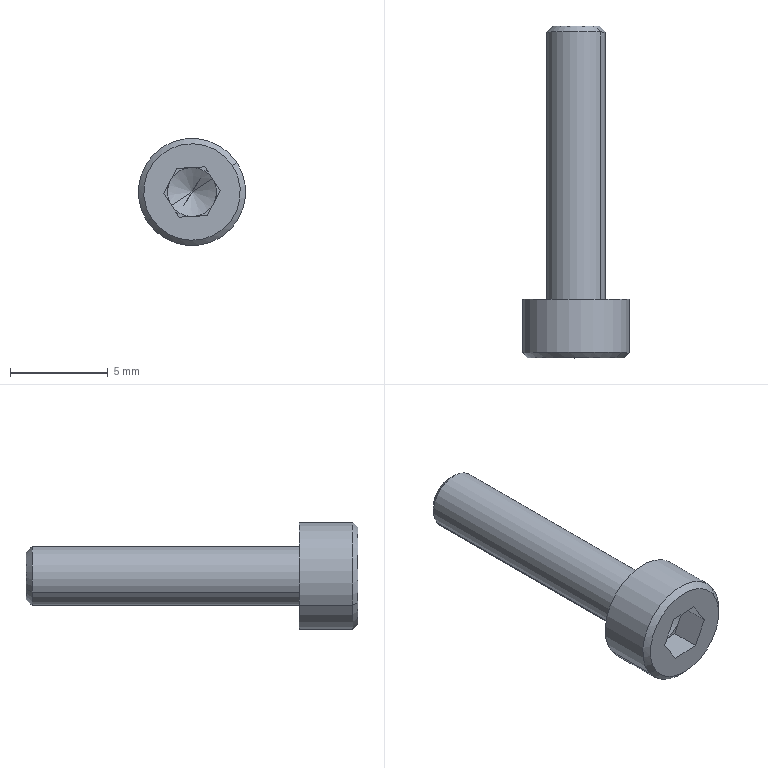Component | SolidWorks | TAC01-M3-L14-1 | 1 solid | 25 faces | box 5.5 x 17 x 5.5 mm | volume 160 mm3 | plane 15 | cone 6 | cylinder 4 | commonest cylinder face diameters 5.5 x2 3 x2
STEP:
#1=CARTESIAN_POINT('',(-2.659,1.633,8.574));
#2=VERTEX_POINT('',#1);
#3=CARTESIAN_POINT('',(-2.7,1.604,8.547));
#4=VERTEX_POINT('',#3);
#5=CARTESIAN_POINT('',(-2.659,1.633,8.574));
#6=DIRECTION('',(-0.725,-0.5,-0.4737));
#7=VECTOR('',#6,39.37);
#8=LINE('',#5,#7);
#9=EDGE_CURVE('',#2,#4,#8,.T.);
#10=ORIENTED_EDGE('',*,*,#9,.F.);
#11=CARTESIAN_POINT('',(-2.618,1.604,8.601));
#12=VERTEX_POINT('',#11);
#13=CARTESIAN_POINT('',(-2.659,1.633,8.574));
#14=DIRECTION('',(0.725,-0.5,0.4737));
#15=VECTOR('',#14,39.37);
#16=LINE('',#13,#15);
#17=EDGE_CURVE('',#2,#12,#16,.T.);
#18=ORIENTED_EDGE('',*,*,#17,.T.);
#19=CARTESIAN_POINT('',(-2.662,1.604,8.623));
#20=VERTEX_POINT('',#19);
#21=CARTESIAN_POINT('',(-2.659,1.604,8.574));
#22=DIRECTION('',(-0.,-1.,0.));
#23=DIRECTION('',(-0.8372,0.,-0.5469));
#24=AXIS2_PLACEMENT_3D('',#21,#22,#23);
#25=CIRCLE('',#24,0.04921);
#26=EDGE_CURVE('',#12,#20,#25,.T.);
#27=ORIENTED_EDGE('',*,*,#26,.T.);
#28=CARTESIAN_POINT('',(-2.703,1.604,8.597));
#29=VERTEX_POINT('',#28);
#30=CARTESIAN_POINT('',(-2.659,1.604,8.574));
#31=DIRECTION('',(-0.,-1.,0.));
#32=DIRECTION('',(-0.8372,0.,-0.5469));
#33=AXIS2_PLACEMENT_3D('',#30,#31,#32);
#34=CIRCLE('',#33,0.04921);
#35=EDGE_CURVE('',#20,#29,#34,.T.);
#36=ORIENTED_EDGE('',*,*,#35,.T.);
#37=CARTESIAN_POINT('',(-2.659,1.604,8.574));
#38=DIRECTION('',(-0.,-1.,0.));
#39=DIRECTION('',(-0.8372,0.,-0.5469));
#40=AXIS2_PLACEMENT_3D('',#37,#38,#39);
#41=CIRCLE('',#40,0.04921);
#42=EDGE_CURVE('',#29,#4,#41,.T.);
#43=ORIENTED_EDGE('',*,*,#42,.T.);
#44=EDGE_LOOP('',(#10,#18,#27,#36,#43));
#45=FACE_OUTER_BOUND('',#44,.T.);
#46=CARTESIAN_POINT('',(-2.659,-37.737,8.574));
#47=DIRECTION('',(-0.,-1.,0.));
#48=DIRECTION('',(-0.8372,0.,-0.5469));
#49=AXIS2_PLACEMENT_3D('',#46,#47,#48);
#50=CONICAL_SURFACE('',#49,68.191,1.047);
#51=ADVANCED_FACE('',(#45),#50,.F.);
#52=CARTESIAN_POINT('',(-2.75,1.663,8.515));
#53=VERTEX_POINT('',#52);
#54=CARTESIAN_POINT('',(-2.568,1.663,8.634));
#55=VERTEX_POINT('',#54);
#56=CARTESIAN_POINT('',(-2.659,1.663,8.574));
#57=DIRECTION('',(-0.,-1.,0.));
#58=DIRECTION('',(-0.8372,0.,-0.5469));
#59=AXIS2_PLACEMENT_3D('',#56,#57,#58);
#60=CIRCLE('',#59,0.1083);
#61=EDGE_CURVE('',#53,#55,#60,.T.);
#62=ORIENTED_EDGE('',*,*,#61,.T.);
#63=CARTESIAN_POINT('',(-2.568,1.556,8.634));
#64=VERTEX_POINT('',#63);
#65=CARTESIAN_POINT('',(-2.568,1.663,8.634));
#66=DIRECTION('',(-0.,-1.,0.));
#67=VECTOR('',#66,39.37);
#68=LINE('',#65,#67);
#69=EDGE_CURVE('',#55,#64,#68,.T.);
#70=ORIENTED_EDGE('',*,*,#69,.T.);
#71=CARTESIAN_POINT('',(-2.75,1.556,8.515));
#72=VERTEX_POINT('',#71);
#73=CARTESIAN_POINT('',(-2.659,1.556,8.574));
#74=DIRECTION('',(-0.,-1.,0.));
#75=DIRECTION('',(-0.8372,0.,-0.5469));
#76=AXIS2_PLACEMENT_3D('',#73,#74,#75);
#77=CIRCLE('',#76,0.1083);
#78=EDGE_CURVE('',#72,#64,#77,.T.);
#79=ORIENTED_EDGE('',*,*,#78,.F.);
#80=CARTESIAN_POINT('',(-2.75,1.663,8.515));
#81=DIRECTION('',(-0.,-1.,0.));
#82=VECTOR('',#81,39.37);
#83=LINE('',#80,#82);
#84=EDGE_CURVE('',#53,#72,#83,.T.);
#85=ORIENTED_EDGE('',*,*,#84,.F.);
#86=EDGE_LOOP('',(#62,#70,#79,#85));
#87=FACE_OUTER_BOUND('',#86,.T.);
#88=CARTESIAN_POINT('',(-2.659,1.663,8.574));
#89=DIRECTION('',(-0.,-1.,0.));
#90=DIRECTION('',(-0.8372,0.,-0.5469));
#91=AXIS2_PLACEMENT_3D('',#88,#89,#90);
#92=CYLINDRICAL_SURFACE('',#91,0.1083);
#93=ADVANCED_FACE('',(#87),#92,.T.);
#94=CARTESIAN_POINT('',(-2.74,1.545,8.521));
#95=VERTEX_POINT('',#94);
#96=CARTESIAN_POINT('',(-2.577,1.545,8.628));
#97=VERTEX_POINT('',#96);
#98=CARTESIAN_POINT('',(-2.659,1.545,8.574));
#99=DIRECTION('',(-0.,-1.,0.));
#100=DIRECTION('',(-0.8372,0.,-0.5469));
#101=AXIS2_PLACEMENT_3D('',#98,#99,#100);
#102=CIRCLE('',#101,0.09744);
#103=EDGE_CURVE('',#95,#97,#102,.T.);
#104=ORIENTED_EDGE('',*,*,#103,.F.);
#105=CARTESIAN_POINT('',(-2.75,1.556,8.515));
#106=DIRECTION('',(-0.592,0.7071,-0.3867));
#107=VECTOR('',#106,39.37);
#108=LINE('',#105,#107);
#109=EDGE_CURVE('',#95,#72,#108,.T.);
#110=ORIENTED_EDGE('',*,*,#109,.T.);
#111=ORIENTED_EDGE('',*,*,#78,.T.);
#112=CARTESIAN_POINT('',(-2.568,1.556,8.634));
#113=DIRECTION('',(0.592,0.7071,0.3867));
#114=VECTOR('',#113,39.37);
#115=LINE('',#112,#114);
#116=EDGE_CURVE('',#97,#64,#115,.T.);
#117=ORIENTED_EDGE('',*,*,#116,.F.);
#118=EDGE_LOOP('',(#104,#110,#111,#117));
#119=FACE_OUTER_BOUND('',#118,.T.);
#120=CARTESIAN_POINT('',(-2.659,1.556,8.574));
#121=DIRECTION('',(0.,1.,-0.));
#122=DIRECTION('',(0.8372,-0.,0.5469));
#123=AXIS2_PLACEMENT_3D('',#120,#121,#122);
#124=CONICAL_SURFACE('',#123,0.1083,0.7854);
#125=ADVANCED_FACE('',(#119),#124,.T.);
#126=CARTESIAN_POINT('',(-2.698,2.215,8.549));
#127=VERTEX_POINT('',#126);
#128=CARTESIAN_POINT('',(-2.62,2.215,8.6));
#129=VERTEX_POINT('',#128);
#130=CARTESIAN_POINT('',(-2.659,2.215,8.574));
#131=DIRECTION('',(-0.,-1.,0.));
#132=DIRECTION('',(-0.8372,0.,-0.5469));
#133=AXIS2_PLACEMENT_3D('',#130,#131,#132);
#134=CIRCLE('',#133,0.04699);
#135=EDGE_CURVE('',#127,#129,#134,.T.);
#136=ORIENTED_EDGE('',*,*,#135,.T.);
#137=CARTESIAN_POINT('',(-2.609,2.202,8.607));
#138=VERTEX_POINT('',#137);
#139=CARTESIAN_POINT('',(-2.62,2.215,8.6));
#140=DIRECTION('',(0.592,-0.7071,0.3867));
#141=VECTOR('',#140,39.37);
#142=LINE('',#139,#141);
#143=EDGE_CURVE('',#129,#138,#142,.T.);
#144=ORIENTED_EDGE('',*,*,#143,.T.);
#145=CARTESIAN_POINT('',(-2.708,2.202,8.542));
#146=VERTEX_POINT('',#145);
#147=CARTESIAN_POINT('',(-2.659,2.202,8.574));
#148=DIRECTION('',(-0.,-1.,0.));
#149=DIRECTION('',(-0.8372,0.,-0.5469));
#150=AXIS2_PLACEMENT_3D('',#147,#148,#149);
#151=CIRCLE('',#150,0.05906);
#152=EDGE_CURVE('',#146,#138,#151,.T.);
#153=ORIENTED_EDGE('',*,*,#152,.F.);
#154=CARTESIAN_POINT('',(-2.698,2.215,8.549));
#155=DIRECTION('',(-0.592,-0.7071,-0.3867));
#156=VECTOR('',#155,39.37);
#157=LINE('',#154,#156);
#158=EDGE_CURVE('',#127,#146,#157,.T.);
#159=ORIENTED_EDGE('',*,*,#158,.F.);
#160=EDGE_LOOP('',(#136,#144,#153,#159));
#161=FACE_OUTER_BOUND('',#160,.T.);
#162=CARTESIAN_POINT('',(-2.659,2.215,8.574));
#163=DIRECTION('',(-0.,-1.,0.));
#164=DIRECTION('',(-0.8372,0.,-0.5469));
#165=AXIS2_PLACEMENT_3D('',#162,#163,#164);
#166=CONICAL_SURFACE('',#165,0.04699,0.7854);
#167=ADVANCED_FACE('',(#161),#166,.T.);
#168=ORIENTED_EDGE('',*,*,#152,.T.);
#169=CARTESIAN_POINT('',(-2.609,1.663,8.607));
#170=VERTEX_POINT('',#169);
#171=CARTESIAN_POINT('',(-2.609,2.215,8.607));
#172=DIRECTION('',(-0.,-1.,0.));
#173=VECTOR('',#172,39.37);
#174=LINE('',#171,#173);
#175=EDGE_CURVE('',#138,#170,#174,.T.);
#176=ORIENTED_EDGE('',*,*,#175,.T.);
#177=CARTESIAN_POINT('',(-2.708,1.663,8.542));
#178=VERTEX_POINT('',#177);
#179=CARTESIAN_POINT('',(-2.659,1.663,8.574));
#180=DIRECTION('',(-0.,-1.,0.));
#181=DIRECTION('',(-0.8372,0.,-0.5469));
#182=AXIS2_PLACEMENT_3D('',#179,#180,#181);
#183=CIRCLE('',#182,0.05906);
#184=EDGE_CURVE('',#178,#170,#183,.T.);
#185=ORIENTED_EDGE('',*,*,#184,.F.);
#186=CARTESIAN_POINT('',(-2.708,2.215,8.542));
#187=DIRECTION('',(-0.,-1.,0.));
#188=VECTOR('',#187,39.37);
#189=LINE('',#186,#188);
#190=EDGE_CURVE('',#146,#178,#189,.T.);
#191=ORIENTED_EDGE('',*,*,#190,.F.);
#192=EDGE_LOOP('',(#168,#176,#185,#191));
#193=FACE_OUTER_BOUND('',#192,.T.);
#194=CARTESIAN_POINT('',(-2.659,2.215,8.574));
#195=DIRECTION('',(-0.,-1.,0.));
#196=DIRECTION('',(-0.8372,0.,-0.5469));
#197=AXIS2_PLACEMENT_3D('',#194,#195,#196);
#198=CYLINDRICAL_SURFACE('',#197,0.05906);
#199=ADVANCED_FACE('',(#193),#198,.T.);
#200=CARTESIAN_POINT('',(-2.656,1.604,8.525));
#201=VERTEX_POINT('',#200);
#202=CARTESIAN_POINT('',(-2.659,1.604,8.574));
#203=DIRECTION('',(-0.,-1.,0.));
#204=DIRECTION('',(-0.8372,0.,-0.5469));
#205=AXIS2_PLACEMENT_3D('',#202,#203,#204);
#206=CIRCLE('',#205,0.04921);
#207=EDGE_CURVE('',#4,#201,#206,.T.);
#208=ORIENTED_EDGE('',*,*,#207,.F.);
#209=CARTESIAN_POINT('',(-2.685,1.604,8.524));
#210=VERTEX_POINT('',#209);
#211=CARTESIAN_POINT('',(-2.716,1.604,8.571));
#212=DIRECTION('',(0.5469,-0.,-0.8372));
#213=VECTOR('',#212,39.37);
#214=LINE('',#211,#213);
#215=EDGE_CURVE('',#4,#210,#214,.T.);
#216=ORIENTED_EDGE('',*,*,#215,.T.);
#217=CARTESIAN_POINT('',(-2.685,1.604,8.524));
#218=DIRECTION('',(0.9985,-0.,0.05508));
#219=VECTOR('',#218,39.37);
#220=LINE('',#217,#219);
#221=EDGE_CURVE('',#210,#201,#220,.T.);
#222=ORIENTED_EDGE('',*,*,#221,.T.);
#223=EDGE_LOOP('',(#208,#216,#222));
#224=FACE_OUTER_BOUND('',#223,.T.);
#225=CARTESIAN_POINT('',(-2.659,1.604,8.574));
#226=DIRECTION('',(-0.,-1.,0.));
#227=DIRECTION('',(-0.8372,0.,-0.5469));
#228=AXIS2_PLACEMENT_3D('',#225,#226,#227);
#229=PLANE('',#228);
#230=ADVANCED_FACE('',(#224),#229,.T.);
#231=CARTESIAN_POINT('',(-2.615,1.604,8.552));
#232=VERTEX_POINT('',#231);
#233=CARTESIAN_POINT('',(-2.659,1.604,8.574));
#234=DIRECTION('',(-0.,-1.,0.));
#235=DIRECTION('',(-0.8372,0.,-0.5469));
#236=AXIS2_PLACEMENT_3D('',#233,#234,#235);
#237=CIRCLE('',#236,0.04921);
#238=EDGE_CURVE('',#201,#232,#237,.T.);
#239=ORIENTED_EDGE('',*,*,#238,.F.);
#240=CARTESIAN_POINT('',(-2.628,1.604,8.527));
#241=VERTEX_POINT('',#240);
#242=CARTESIAN_POINT('',(-2.685,1.604,8.524));
#243=DIRECTION('',(0.9985,-0.,0.05508));
#244=VECTOR('',#243,39.37);
#245=LINE('',#242,#244);
#246=EDGE_CURVE('',#201,#241,#245,.T.);
#247=ORIENTED_EDGE('',*,*,#246,.T.);
#248=CARTESIAN_POINT('',(-2.628,1.604,8.527));
#249=DIRECTION('',(0.4515,-0.,0.8923));
#250=VECTOR('',#249,39.37);
#251=LINE('',#248,#250);
#252=EDGE_CURVE('',#241,#232,#251,.T.);
#253=ORIENTED_EDGE('',*,*,#252,.T.);
#254=EDGE_LOOP('',(#239,#247,#253));
#255=FACE_OUTER_BOUND('',#254,.T.);
#256=CARTESIAN_POINT('',(-2.659,1.604,8.574));
#257=DIRECTION('',(-0.,-1.,0.));
#258=DIRECTION('',(-0.8372,0.,-0.5469));
#259=AXIS2_PLACEMENT_3D('',#256,#257,#258);
#260=PLANE('',#259);
#261=ADVANCED_FACE('',(#255),#260,.T.);
#262=CARTESIAN_POINT('',(-2.659,1.604,8.574));
#263=DIRECTION('',(-0.,-1.,0.));
#264=DIRECTION('',(-0.8372,0.,-0.5469));
#265=AXIS2_PLACEMENT_3D('',#262,#263,#264);
#266=CIRCLE('',#265,0.04921);
#267=EDGE_CURVE('',#232,#12,#266,.T.);
#268=ORIENTED_EDGE('',*,*,#267,.F.);
#269=CARTESIAN_POINT('',(-2.602,1.604,8.577));
#270=VERTEX_POINT('',#269);
#271=CARTESIAN_POINT('',(-2.628,1.604,8.527));
#272=DIRECTION('',(0.4515,-0.,0.8923));
#273=VECTOR('',#272,39.37);
#274=LINE('',#271,#273);
#275=EDGE_CURVE('',#232,#270,#274,.T.);
#276=ORIENTED_EDGE('',*,*,#275,.T.);
#277=CARTESIAN_POINT('',(-2.602,1.604,8.577));
#278=DIRECTION('',(-0.5469,0.,0.8372));
#279=VECTOR('',#278,39.37);
#280=LINE('',#277,#279);
#281=EDGE_CURVE('',#270,#12,#280,.T.);
#282=ORIENTED_EDGE('',*,*,#281,.T.);
#283=EDGE_LOOP('',(#268,#276,#282));
#284=FACE_OUTER_BOUND('',#283,.T.);
#285=CARTESIAN_POINT('',(-2.659,1.604,8.574));
#286=DIRECTION('',(-0.,-1.,0.));
#287=DIRECTION('',(-0.8372,0.,-0.5469));
#288=AXIS2_PLACEMENT_3D('',#285,#286,#287);
#289=PLANE('',#288);
#290=ADVANCED_FACE('',(#284),#289,.T.);
#291=ORIENTED_EDGE('',*,*,#26,.F.);
#292=CARTESIAN_POINT('',(-2.633,1.604,8.625));
#293=VERTEX_POINT('',#292);
#294=CARTESIAN_POINT('',(-2.602,1.604,8.577));
#295=DIRECTION('',(-0.5469,0.,0.8372));
#296=VECTOR('',#295,39.37);
#297=LINE('',#294,#296);
#298=EDGE_CURVE('',#12,#293,#297,.T.);
#299=ORIENTED_EDGE('',*,*,#298,.T.);
#300=CARTESIAN_POINT('',(-2.633,1.604,8.625));
#301=DIRECTION('',(-0.9985,0.,-0.05508));
#302=VECTOR('',#301,39.37);
#303=LINE('',#300,#302);
#304=EDGE_CURVE('',#293,#20,#303,.T.);
#305=ORIENTED_EDGE('',*,*,#304,.T.);
#306=EDGE_LOOP('',(#291,#299,#305));
#307=FACE_OUTER_BOUND('',#306,.T.);
#308=CARTESIAN_POINT('',(-2.659,1.604,8.574));
#309=DIRECTION('',(-0.,-1.,0.));
#310=DIRECTION('',(-0.8372,0.,-0.5469));
#311=AXIS2_PLACEMENT_3D('',#308,#309,#310);
#312=PLANE('',#311);
#313=ADVANCED_FACE('',(#307),#312,.T.);
#314=ORIENTED_EDGE('',*,*,#35,.F.);
#315=CARTESIAN_POINT('',(-2.69,1.604,8.622));
#316=VERTEX_POINT('',#315);
#317=CARTESIAN_POINT('',(-2.633,1.604,8.625));
#318=DIRECTION('',(-0.9985,0.,-0.05508));
#319=VECTOR('',#318,39.37);
#320=LINE('',#317,#319);
#321=EDGE_CURVE('',#20,#316,#320,.T.);
#322=ORIENTED_EDGE('',*,*,#321,.T.);
#323=CARTESIAN_POINT('',(-2.69,1.604,8.622));
#324=DIRECTION('',(-0.4515,0.,-0.8923));
#325=VECTOR('',#324,39.37);
#326=LINE('',#323,#325);
#327=EDGE_CURVE('',#316,#29,#326,.T.);
#328=ORIENTED_EDGE('',*,*,#327,.T.);
#329=EDGE_LOOP('',(#314,#322,#328));
#330=FACE_OUTER_BOUND('',#329,.T.);
#331=CARTESIAN_POINT('',(-2.659,1.604,8.574));
#332=DIRECTION('',(-0.,-1.,0.));
#333=DIRECTION('',(-0.8372,0.,-0.5469));
#334=AXIS2_PLACEMENT_3D('',#331,#332,#333);
#335=PLANE('',#334);
#336=ADVANCED_FACE('',(#330),#335,.T.);
#337=ORIENTED_EDGE('',*,*,#175,.F.);
#338=CARTESIAN_POINT('',(-2.659,2.202,8.574));
#339=DIRECTION('',(-0.,-1.,0.));
#340=DIRECTION('',(-0.8372,0.,-0.5469));
#341=AXIS2_PLACEMENT_3D('',#338,#339,#340);
#342=CIRCLE('',#341,0.05906);
#343=EDGE_CURVE('',#138,#146,#342,.T.);
#344=ORIENTED_EDGE('',*,*,#343,.T.);
#345=ORIENTED_EDGE('',*,*,#190,.T.);
#346=CARTESIAN_POINT('',(-2.659,1.663,8.574));
#347=DIRECTION('',(-0.,-1.,0.));
#348=DIRECTION('',(-0.8372,0.,-0.5469));
#349=AXIS2_PLACEMENT_3D('',#346,#347,#348);
#350=CIRCLE('',#349,0.05906);
#351=EDGE_CURVE('',#170,#178,#350,.T.);
#352=ORIENTED_EDGE('',*,*,#351,.F.);
#353=EDGE_LOOP('',(#337,#344,#345,#352));
#354=FACE_OUTER_BOUND('',#353,.T.);
#355=CARTESIAN_POINT('',(-2.659,2.215,8.574));
#356=DIRECTION('',(-0.,-1.,0.));
#357=DIRECTION('',(-0.8372,0.,-0.5469));
#358=AXIS2_PLACEMENT_3D('',#355,#356,#357);
#359=CYLINDRICAL_SURFACE('',#358,0.05906);
#360=ADVANCED_FACE('',(#354),#359,.T.);
#361=ORIENTED_EDGE('',*,*,#143,.F.);
#362=CARTESIAN_POINT('',(-2.659,2.215,8.574));
#363=DIRECTION('',(-0.,-1.,0.));
#364=DIRECTION('',(-0.8372,0.,-0.5469));
#365=AXIS2_PLACEMENT_3D('',#362,#363,#364);
#366=CIRCLE('',#365,0.04699);
#367=EDGE_CURVE('',#129,#127,#366,.T.);
#368=ORIENTED_EDGE('',*,*,#367,.T.);
#369=ORIENTED_EDGE('',*,*,#158,.T.);
#370=ORIENTED_EDGE('',*,*,#343,.F.);
#371=EDGE_LOOP('',(#361,#368,#369,#370));
#372=FACE_OUTER_BOUND('',#371,.T.);
#373=CARTESIAN_POINT('',(-2.659,2.215,8.574));
#374=DIRECTION('',(-0.,-1.,0.));
#375=DIRECTION('',(-0.8372,0.,-0.5469));
#376=AXIS2_PLACEMENT_3D('',#373,#374,#375);
#377=CONICAL_SURFACE('',#376,0.04699,0.7854);
#378=ADVANCED_FACE('',(#372),#377,.T.);
#379=ORIENTED_EDGE('',*,*,#135,.F.);
#380=ORIENTED_EDGE('',*,*,#367,.F.);
#381=EDGE_LOOP('',(#379,#380));
#382=FACE_OUTER_BOUND('',#381,.T.);
#383=CARTESIAN_POINT('',(-2.633,2.215,8.535));
#384=DIRECTION('',(-0.,-1.,0.));
#385=DIRECTION('',(-0.8372,0.,-0.5469));
#386=AXIS2_PLACEMENT_3D('',#383,#384,#385);
#387=PLANE('',#386);
#388=ADVANCED_FACE('',(#382),#387,.F.);
#389=CARTESIAN_POINT('',(-2.69,1.545,8.622));
#390=VERTEX_POINT('',#389);
#391=CARTESIAN_POINT('',(-2.716,1.545,8.571));
#392=VERTEX_POINT('',#391);
#393=CARTESIAN_POINT('',(-2.69,1.545,8.622));
#394=DIRECTION('',(-0.4515,0.,-0.8923));
#395=VECTOR('',#394,39.37);
#396=LINE('',#393,#395);
#397=EDGE_CURVE('',#390,#392,#396,.T.);
#398=ORIENTED_EDGE('',*,*,#397,.F.);
#399=CARTESIAN_POINT('',(-2.633,1.545,8.625));
#400=VERTEX_POINT('',#399);
#401=CARTESIAN_POINT('',(-2.633,1.545,8.625));
#402=DIRECTION('',(-0.9985,0.,-0.05508));
#403=VECTOR('',#402,39.37);
#404=LINE('',#401,#403);
#405=EDGE_CURVE('',#400,#390,#404,.T.);
#406=ORIENTED_EDGE('',*,*,#405,.F.);
#407=CARTESIAN_POINT('',(-2.602,1.545,8.577));
#408=VERTEX_POINT('',#407);
#409=CARTESIAN_POINT('',(-2.602,1.545,8.577));
#410=DIRECTION('',(-0.5469,0.,0.8372));
#411=VECTOR('',#410,39.37);
#412=LINE('',#409,#411);
#413=EDGE_CURVE('',#408,#400,#412,.T.);
#414=ORIENTED_EDGE('',*,*,#413,.F.);
#415=CARTESIAN_POINT('',(-2.628,1.545,8.527));
#416=VERTEX_POINT('',#415);
#417=CARTESIAN_POINT('',(-2.628,1.545,8.527));
#418=DIRECTION('',(0.4515,-0.,0.8923));
#419=VECTOR('',#418,39.37);
#420=LINE('',#417,#419);
#421=EDGE_CURVE('',#416,#408,#420,.T.);
#422=ORIENTED_EDGE('',*,*,#421,.F.);
#423=CARTESIAN_POINT('',(-2.685,1.545,8.524));
#424=VERTEX_POINT('',#423);
#425=CARTESIAN_POINT('',(-2.685,1.545,8.524));
#426=DIRECTION('',(0.9985,-0.,0.05508));
#427=VECTOR('',#426,39.37);
#428=LINE('',#425,#427);
#429=EDGE_CURVE('',#424,#416,#428,.T.);
#430=ORIENTED_EDGE('',*,*,#429,.F.);
#431=CARTESIAN_POINT('',(-2.716,1.545,8.571));
#432=DIRECTION('',(0.5469,-0.,-0.8372));
#433=VECTOR('',#432,39.37);
#434=LINE('',#431,#433);
#435=EDGE_CURVE('',#392,#424,#434,.T.);
#436=ORIENTED_EDGE('',*,*,#435,.F.);
#437=EDGE_LOOP('',(#398,#406,#414,#422,#430,#436));
#438=FACE_BOUND('',#437,.T.);
#439=CARTESIAN_POINT('',(-2.659,1.545,8.574));
#440=DIRECTION('',(-0.,-1.,0.));
#441=DIRECTION('',(-0.8372,0.,-0.5469));
#442=AXIS2_PLACEMENT_3D('',#439,#440,#441);
#443=CIRCLE('',#442,0.09744);
#444=EDGE_CURVE('',#97,#95,#443,.T.);
#445=ORIENTED_EDGE('',*,*,#444,.T.);
#446=ORIENTED_EDGE('',*,*,#103,.T.);
#447=EDGE_LOOP('',(#445,#446));
#448=FACE_OUTER_BOUND('',#447,.T.);
#449=CARTESIAN_POINT('',(-2.659,1.545,8.574));
#450=DIRECTION('',(0.,1.,0.));
#451=DIRECTION('',(0.8372,-0.,0.5469));
#452=AXIS2_PLACEMENT_3D('',#449,#450,#451);
#453=PLANE('',#452);
#454=ADVANCED_FACE('',(#438,#448),#453,.F.);
#455=ORIENTED_EDGE('',*,*,#109,.F.);
#456=ORIENTED_EDGE('',*,*,#444,.F.);
#457=ORIENTED_EDGE('',*,*,#116,.T.);
#458=CARTESIAN_POINT('',(-2.659,1.556,8.574));
#459=DIRECTION('',(-0.,-1.,0.));
#460=DIRECTION('',(-0.8372,0.,-0.5469));
#461=AXIS2_PLACEMENT_3D('',#458,#459,#460);
#462=CIRCLE('',#461,0.1083);
#463=EDGE_CURVE('',#64,#72,#462,.T.);
#464=ORIENTED_EDGE('',*,*,#463,.T.);
#465=EDGE_LOOP('',(#455,#456,#457,#464));
#466=FACE_OUTER_BOUND('',#465,.T.);
#467=CARTESIAN_POINT('',(-2.659,1.556,8.574));
#468=DIRECTION('',(0.,1.,-0.));
#469=DIRECTION('',(0.8372,-0.,0.5469));
#470=AXIS2_PLACEMENT_3D('',#467,#468,#469);
#471=CONICAL_SURFACE('',#470,0.1083,0.7854);
#472=ADVANCED_FACE('',(#466),#471,.T.);
#473=ORIENTED_EDGE('',*,*,#69,.F.);
#474=CARTESIAN_POINT('',(-2.659,1.663,8.574));
#475=DIRECTION('',(-0.,-1.,0.));
#476=DIRECTION('',(-0.8372,0.,-0.5469));
#477=AXIS2_PLACEMENT_3D('',#474,#475,#476);
#478=CIRCLE('',#477,0.1083);
#479=EDGE_CURVE('',#55,#53,#478,.T.);
#480=ORIENTED_EDGE('',*,*,#479,.T.);
#481=ORIENTED_EDGE('',*,*,#84,.T.);
#482=ORIENTED_EDGE('',*,*,#463,.F.);
#483=EDGE_LOOP('',(#473,#480,#481,#482));
#484=FACE_OUTER_BOUND('',#483,.T.);
#485=CARTESIAN_POINT('',(-2.659,1.663,8.574));
#486=DIRECTION('',(-0.,-1.,0.));
#487=DIRECTION('',(-0.8372,0.,-0.5469));
#488=AXIS2_PLACEMENT_3D('',#485,#486,#487);
#489=CYLINDRICAL_SURFACE('',#488,0.1083);
#490=ADVANCED_FACE('',(#484),#489,.T.);
#491=ORIENTED_EDGE('',*,*,#184,.T.);
#492=ORIENTED_EDGE('',*,*,#351,.T.);
#493=EDGE_LOOP('',(#491,#492));
#494=FACE_BOUND('',#493,.T.);
#495=ORIENTED_EDGE('',*,*,#61,.F.);
#496=ORIENTED_EDGE('',*,*,#479,.F.);
#497=EDGE_LOOP('',(#495,#496));
#498=FACE_OUTER_BOUND('',#497,.T.);
#499=CARTESIAN_POINT('',(-2.6,1.663,8.484));
#500=DIRECTION('',(-0.,-1.,0.));
#501=DIRECTION('',(-0.8372,0.,-0.5469));
#502=AXIS2_PLACEMENT_3D('',#499,#500,#501);
#503=PLANE('',#502);
#504=ADVANCED_FACE('',(#494,#498),#503,.F.);
#505=ORIENTED_EDGE('',*,*,#405,.T.);
#506=CARTESIAN_POINT('',(-2.69,1.604,8.622));
#507=DIRECTION('',(-0.,-1.,0.));
#508=VECTOR('',#507,39.37);
#509=LINE('',#506,#508);
#510=EDGE_CURVE('',#316,#390,#509,.T.);
#511=ORIENTED_EDGE('',*,*,#510,.F.);
#512=ORIENTED_EDGE('',*,*,#321,.F.);
#513=ORIENTED_EDGE('',*,*,#304,.F.);
#514=CARTESIAN_POINT('',(-2.633,1.604,8.625));
#515=DIRECTION('',(-0.,-1.,0.));
#516=VECTOR('',#515,39.37);
#517=LINE('',#514,#516);
#518=EDGE_CURVE('',#293,#400,#517,.T.);
#519=ORIENTED_EDGE('',*,*,#518,.T.);
#520=EDGE_LOOP('',(#505,#511,#512,#513,#519));
#521=FACE_OUTER_BOUND('',#520,.T.);
#522=CARTESIAN_POINT('',(-2.633,1.604,8.625));
#523=DIRECTION('',(-0.05508,0.,0.9985));
#524=DIRECTION('',(-0.9985,0.,-0.05508));
#525=AXIS2_PLACEMENT_3D('',#522,#523,#524);
#526=PLANE('',#525);
#527=ADVANCED_FACE('',(#521),#526,.F.);
#528=ORIENTED_EDGE('',*,*,#413,.T.);
#529=ORIENTED_EDGE('',*,*,#518,.F.);
#530=ORIENTED_EDGE('',*,*,#298,.F.);
#531=ORIENTED_EDGE('',*,*,#281,.F.);
#532=CARTESIAN_POINT('',(-2.602,1.604,8.577));
#533=DIRECTION('',(-0.,-1.,0.));
#534=VECTOR('',#533,39.37);
#535=LINE('',#532,#534);
#536=EDGE_CURVE('',#270,#408,#535,.T.);
#537=ORIENTED_EDGE('',*,*,#536,.T.);
#538=EDGE_LOOP('',(#528,#529,#530,#531,#537));
#539=FACE_OUTER_BOUND('',#538,.T.);
#540=CARTESIAN_POINT('',(-2.602,1.604,8.577));
#541=DIRECTION('',(0.8372,-0.,0.5469));
#542=DIRECTION('',(-0.,-1.,0.));
#543=AXIS2_PLACEMENT_3D('',#540,#541,#542);
#544=PLANE('',#543);
#545=ADVANCED_FACE('',(#539),#544,.F.);
#546=ORIENTED_EDGE('',*,*,#421,.T.);
#547=ORIENTED_EDGE('',*,*,#536,.F.);
#548=ORIENTED_EDGE('',*,*,#275,.F.);
#549=ORIENTED_EDGE('',*,*,#252,.F.);
#550=CARTESIAN_POINT('',(-2.628,1.604,8.527));
#551=DIRECTION('',(-0.,-1.,0.));
#552=VECTOR('',#551,39.37);
#553=LINE('',#550,#552);
#554=EDGE_CURVE('',#241,#416,#553,.T.);
#555=ORIENTED_EDGE('',*,*,#554,.T.);
#556=EDGE_LOOP('',(#546,#547,#548,#549,#555));
#557=FACE_OUTER_BOUND('',#556,.T.);
#558=CARTESIAN_POINT('',(-2.628,1.604,8.527));
#559=DIRECTION('',(0.8923,-0.,-0.4515));
#560=DIRECTION('',(0.4515,-0.,0.8923));
#561=AXIS2_PLACEMENT_3D('',#558,#559,#560);
#562=PLANE('',#561);
#563=ADVANCED_FACE('',(#557),#562,.F.);
#564=ORIENTED_EDGE('',*,*,#429,.T.);
#565=ORIENTED_EDGE('',*,*,#554,.F.);
#566=ORIENTED_EDGE('',*,*,#246,.F.);
#567=ORIENTED_EDGE('',*,*,#221,.F.);
#568=CARTESIAN_POINT('',(-2.685,1.604,8.524));
#569=DIRECTION('',(-0.,-1.,0.));
#570=VECTOR('',#569,39.37);
#571=LINE('',#568,#570);
#572=EDGE_CURVE('',#210,#424,#571,.T.);
#573=ORIENTED_EDGE('',*,*,#572,.T.);
#574=EDGE_LOOP('',(#564,#565,#566,#567,#573));
#575=FACE_OUTER_BOUND('',#574,.T.);
#576=CARTESIAN_POINT('',(-2.685,1.604,8.524));
#577=DIRECTION('',(0.05508,-0.,-0.9985));
#578=DIRECTION('',(0.9985,-0.,0.05508));
#579=AXIS2_PLACEMENT_3D('',#576,#577,#578);
#580=PLANE('',#579);
#581=ADVANCED_FACE('',(#575),#580,.F.);
#582=ORIENTED_EDGE('',*,*,#435,.T.);
#583=ORIENTED_EDGE('',*,*,#572,.F.);
#584=ORIENTED_EDGE('',*,*,#215,.F.);
#585=CARTESIAN_POINT('',(-2.716,1.604,8.571));
#586=VERTEX_POINT('',#585);
#587=CARTESIAN_POINT('',(-2.716,1.604,8.571));
#588=DIRECTION('',(0.5469,-0.,-0.8372));
#589=VECTOR('',#588,39.37);
#590=LINE('',#587,#589);
#591=EDGE_CURVE('',#586,#4,#590,.T.);
#592=ORIENTED_EDGE('',*,*,#591,.F.);
#593=CARTESIAN_POINT('',(-2.716,1.604,8.571));
#594=DIRECTION('',(-0.,-1.,0.));
#595=VECTOR('',#594,39.37);
#596=LINE('',#593,#595);
#597=EDGE_CURVE('',#586,#392,#596,.T.);
#598=ORIENTED_EDGE('',*,*,#597,.T.);
#599=EDGE_LOOP('',(#582,#583,#584,#592,#598));
#600=FACE_OUTER_BOUND('',#599,.T.);
#601=CARTESIAN_POINT('',(-2.716,1.604,8.571));
#602=DIRECTION('',(-0.8372,0.,-0.5469));
#603=DIRECTION('',(0.,1.,-0.));
#604=AXIS2_PLACEMENT_3D('',#601,#602,#603);
#605=PLANE('',#604);
#606=ADVANCED_FACE('',(#600),#605,.F.);
#607=ORIENTED_EDGE('',*,*,#397,.T.);
#608=ORIENTED_EDGE('',*,*,#597,.F.);
#609=CARTESIAN_POINT('',(-2.69,1.604,8.622));
#610=DIRECTION('',(-0.4515,0.,-0.8923));
#611=VECTOR('',#610,39.37);
#612=LINE('',#609,#611);
#613=EDGE_CURVE('',#29,#586,#612,.T.);
#614=ORIENTED_EDGE('',*,*,#613,.F.);
#615=ORIENTED_EDGE('',*,*,#327,.F.);
#616=ORIENTED_EDGE('',*,*,#510,.T.);
#617=EDGE_LOOP('',(#607,#608,#614,#615,#616));
#618=FACE_OUTER_BOUND('',#617,.T.);
#619=CARTESIAN_POINT('',(-2.69,1.604,8.622));
#620=DIRECTION('',(-0.8923,0.,0.4515));
#621=DIRECTION('',(-0.4515,0.,-0.8923));
#622=AXIS2_PLACEMENT_3D('',#619,#620,#621);
#623=PLANE('',#622);
#624=ADVANCED_FACE('',(#618),#623,.F.);
#625=ORIENTED_EDGE('',*,*,#42,.F.);
#626=ORIENTED_EDGE('',*,*,#613,.T.);
#627=ORIENTED_EDGE('',*,*,#591,.T.);
#628=EDGE_LOOP('',(#625,#626,#627));
#629=FACE_OUTER_BOUND('',#628,.T.);
#630=CARTESIAN_POINT('',(-2.659,1.604,8.574));
#631=DIRECTION('',(-0.,-1.,0.));
#632=DIRECTION('',(-0.8372,0.,-0.5469));
#633=AXIS2_PLACEMENT_3D('',#630,#631,#632);
#634=PLANE('',#633);
#635=ADVANCED_FACE('',(#629),#634,.T.);
#636=ORIENTED_EDGE('',*,*,#17,.F.);
#637=ORIENTED_EDGE('',*,*,#9,.T.);
#638=ORIENTED_EDGE('',*,*,#207,.T.);
#639=ORIENTED_EDGE('',*,*,#238,.T.);
#640=ORIENTED_EDGE('',*,*,#267,.T.);
#641=EDGE_LOOP('',(#636,#637,#638,#639,#640));
#642=FACE_OUTER_BOUND('',#641,.T.);
#643=CARTESIAN_POINT('',(-2.659,-37.737,8.574));
#644=DIRECTION('',(-0.,-1.,0.));
#645=DIRECTION('',(-0.8372,0.,-0.5469));
#646=AXIS2_PLACEMENT_3D('',#643,#644,#645);
#647=CONICAL_SURFACE('',#646,68.191,1.047);
#648=ADVANCED_FACE('',(#642),#647,.F.);
#649=CLOSED_SHELL('',(#51,#93,#125,#167,#199,#230,#261,#290,#313,#336,#360,#378,#388,#454,#472,#490,#504,#527,#545,#563,#581,#606,#624,#635,#648));
#650=MANIFOLD_SOLID_BREP('',#649);
#651=CARTESIAN_POINT('',(0.,0.,0.));
#652=DIRECTION('',(0.,0.,1.));
#653=DIRECTION('',(1.,0.,0.));
#654=AXIS2_PLACEMENT_3D('',#651,#652,#653);
#655=(LENGTH_UNIT()NAMED_UNIT(*)SI_UNIT($,.METRE.));
#656=LENGTH_MEASURE_WITH_UNIT(LENGTH_MEASURE(0.0254),#655);
#657=DIMENSIONAL_EXPONENTS(1.,0.,0.,0.,0.,0.,0.);
#658=(CONVERSION_BASED_UNIT('',#656)LENGTH_UNIT()NAMED_UNIT(#657));
#659=UNCERTAINTY_MEASURE_WITH_UNIT(LENGTH_MEASURE(0.00001),#658,'','');
#660=(NAMED_UNIT(*)PLANE_ANGLE_UNIT()SI_UNIT($,.RADIAN.));
#661=(NAMED_UNIT(*)SI_UNIT($,.STERADIAN.)SOLID_ANGLE_UNIT());
#662=(GEOMETRIC_REPRESENTATION_CONTEXT(3)GLOBAL_UNCERTAINTY_ASSIGNED_CONTEXT((#659))GLOBAL_UNIT_ASSIGNED_CONTEXT((#658,#660,#661))REPRESENTATION_CONTEXT('',''));
#663=ADVANCED_BREP_SHAPE_REPRESENTATION('',(#650,#654),#662);
#664=COLOUR_RGB('',0.7922,0.8196,0.9333);
#665=FILL_AREA_STYLE_COLOUR('',#664);
#666=FILL_AREA_STYLE('',(#665));
#667=SURFACE_STYLE_FILL_AREA(#666);
#668=SURFACE_SIDE_STYLE('',(#667));
#669=SURFACE_STYLE_USAGE(.BOTH.,#668);
#670=PRESENTATION_STYLE_ASSIGNMENT((#669));
#671=STYLED_ITEM('',(#670),#650);
#672=PRESENTATION_LAYER_ASSIGNMENT('','',(#671));
#673=(LENGTH_UNIT()NAMED_UNIT(*)SI_UNIT($,.METRE.));
#674=LENGTH_MEASURE_WITH_UNIT(LENGTH_MEASURE(0.0254),#673);
#675=DIMENSIONAL_EXPONENTS(1.,0.,0.,0.,0.,0.,0.);
#676=(CONVERSION_BASED_UNIT('',#674)LENGTH_UNIT()NAMED_UNIT(#675));
#677=UNCERTAINTY_MEASURE_WITH_UNIT(LENGTH_MEASURE(0.00001),#676,'','');
#678=(NAMED_UNIT(*)PLANE_ANGLE_UNIT()SI_UNIT($,.RADIAN.));
#679=(NAMED_UNIT(*)SI_UNIT($,.STERADIAN.)SOLID_ANGLE_UNIT());
#680=(GEOMETRIC_REPRESENTATION_CONTEXT(3)GLOBAL_UNCERTAINTY_ASSIGNED_CONTEXT((#677))GLOBAL_UNIT_ASSIGNED_CONTEXT((#676,#678,#679))REPRESENTATION_CONTEXT('',''));
#681=MECHANICAL_DESIGN_GEOMETRIC_PRESENTATION_REPRESENTATION('',(#671),#680);